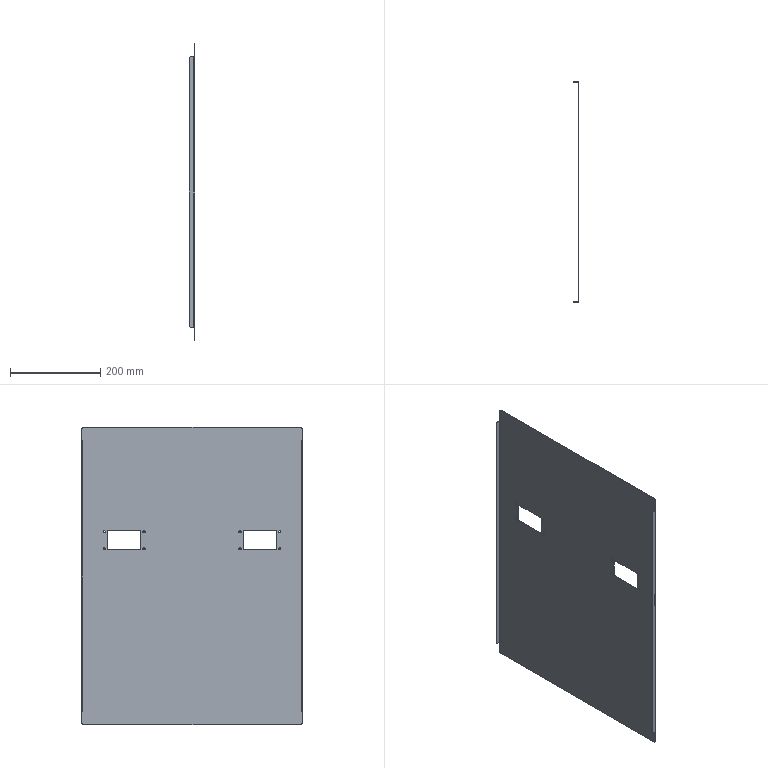Component | SolidWorks | ThreeLowRackSidePlate1-2 | 1 solid | 70 faces | volume 392300 mm3 | plane 46 | cylinder 24 | commonest cylinder face diameters 5 x16 10 x4 3.873 x2 1.473 x2 | material AISI 304